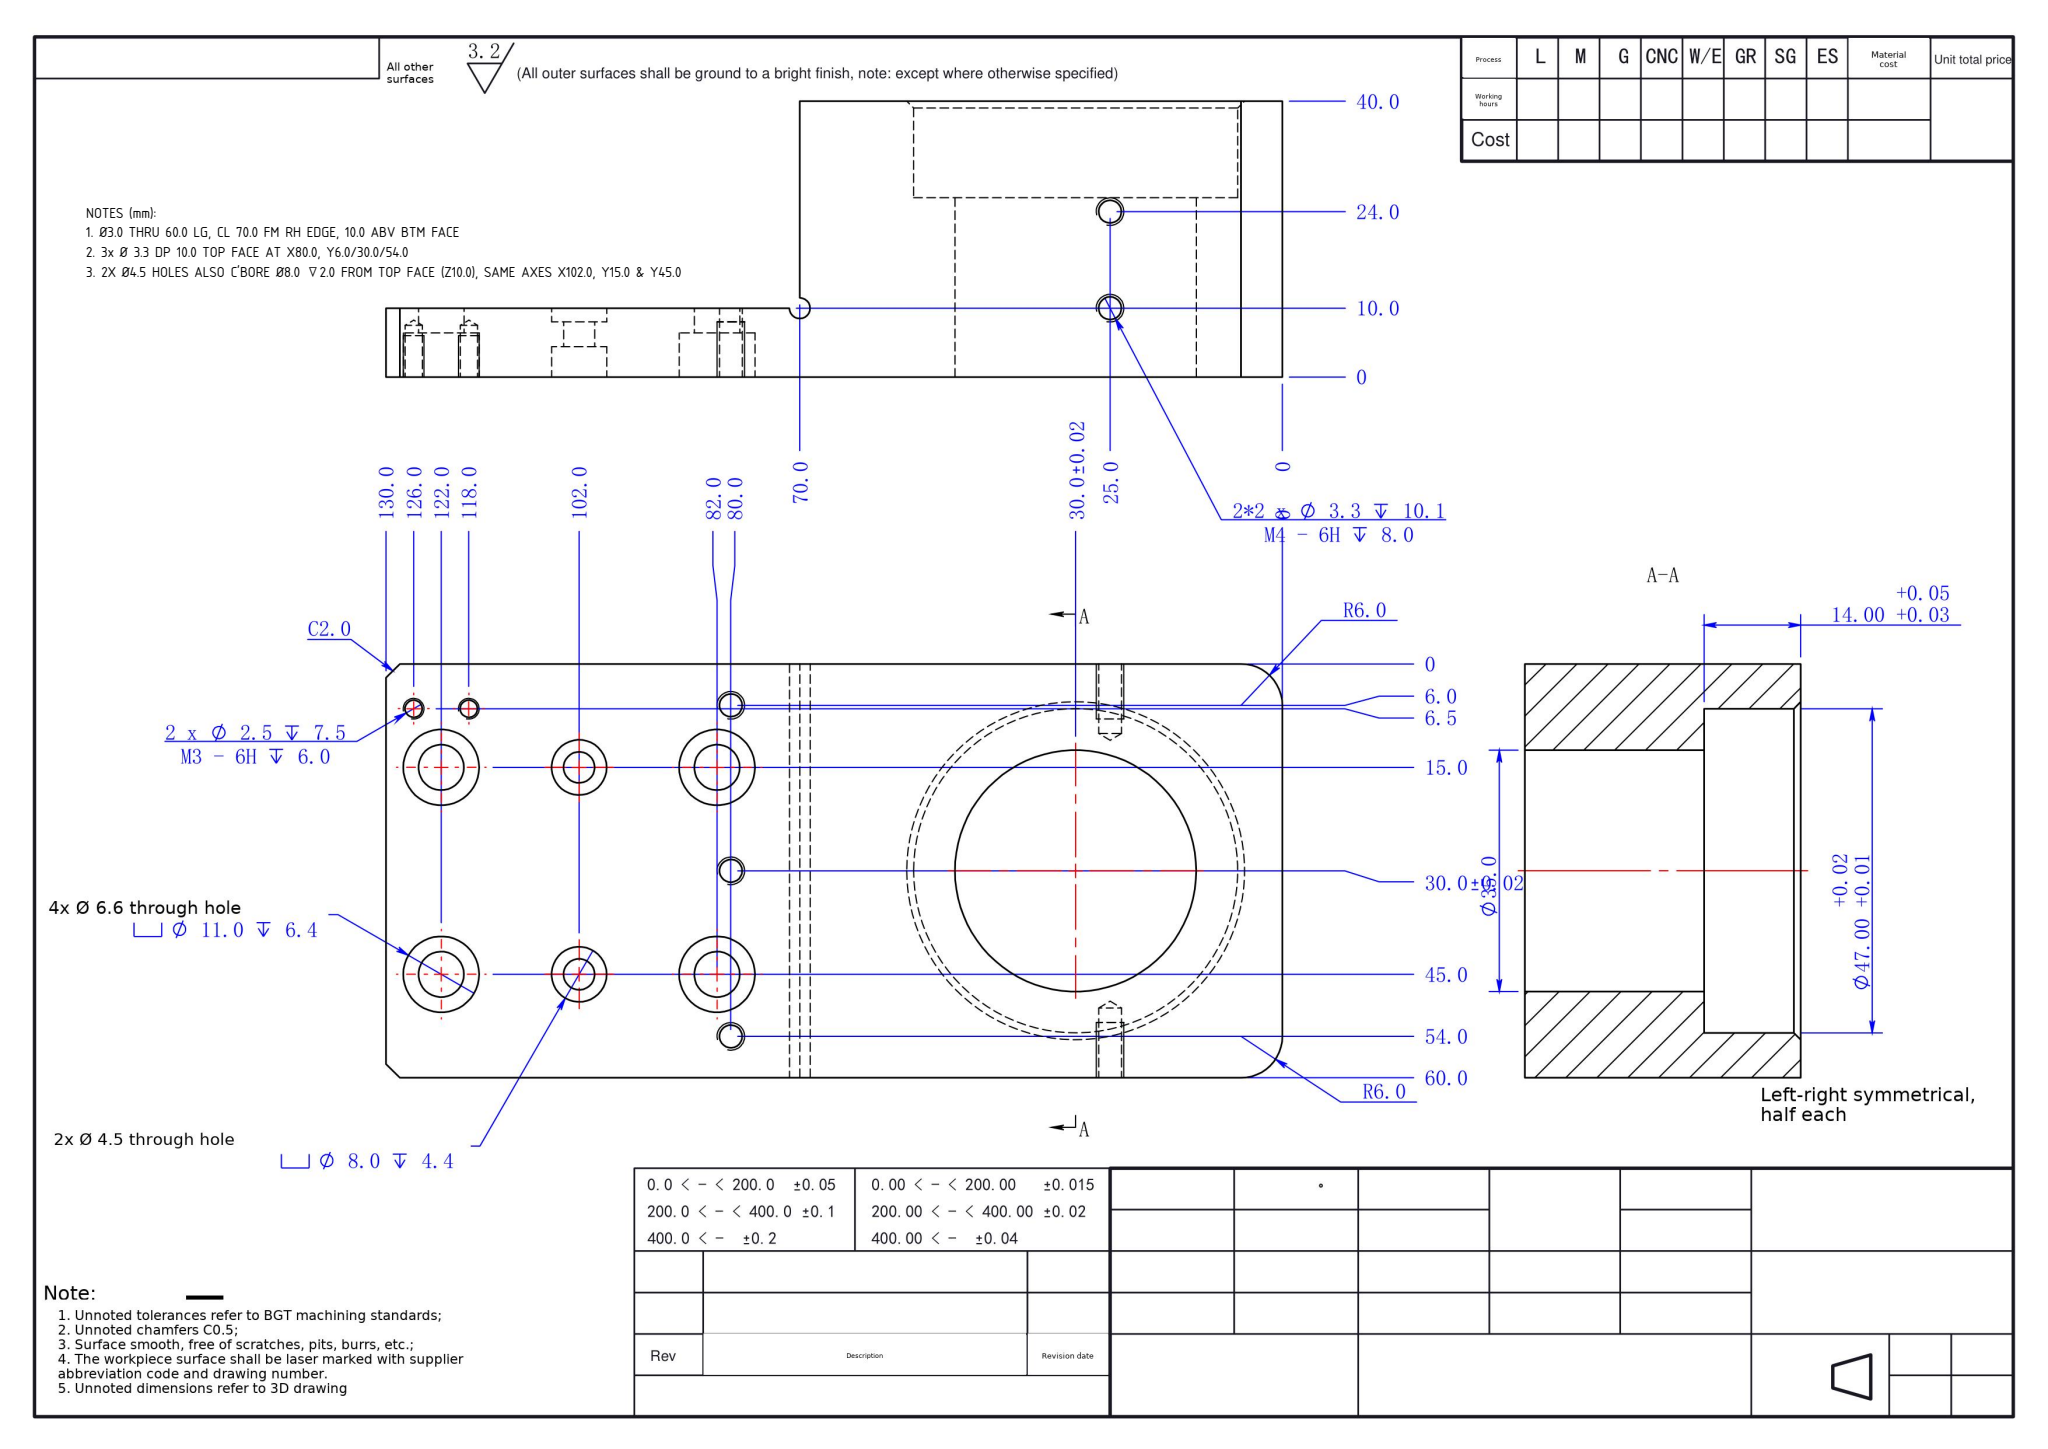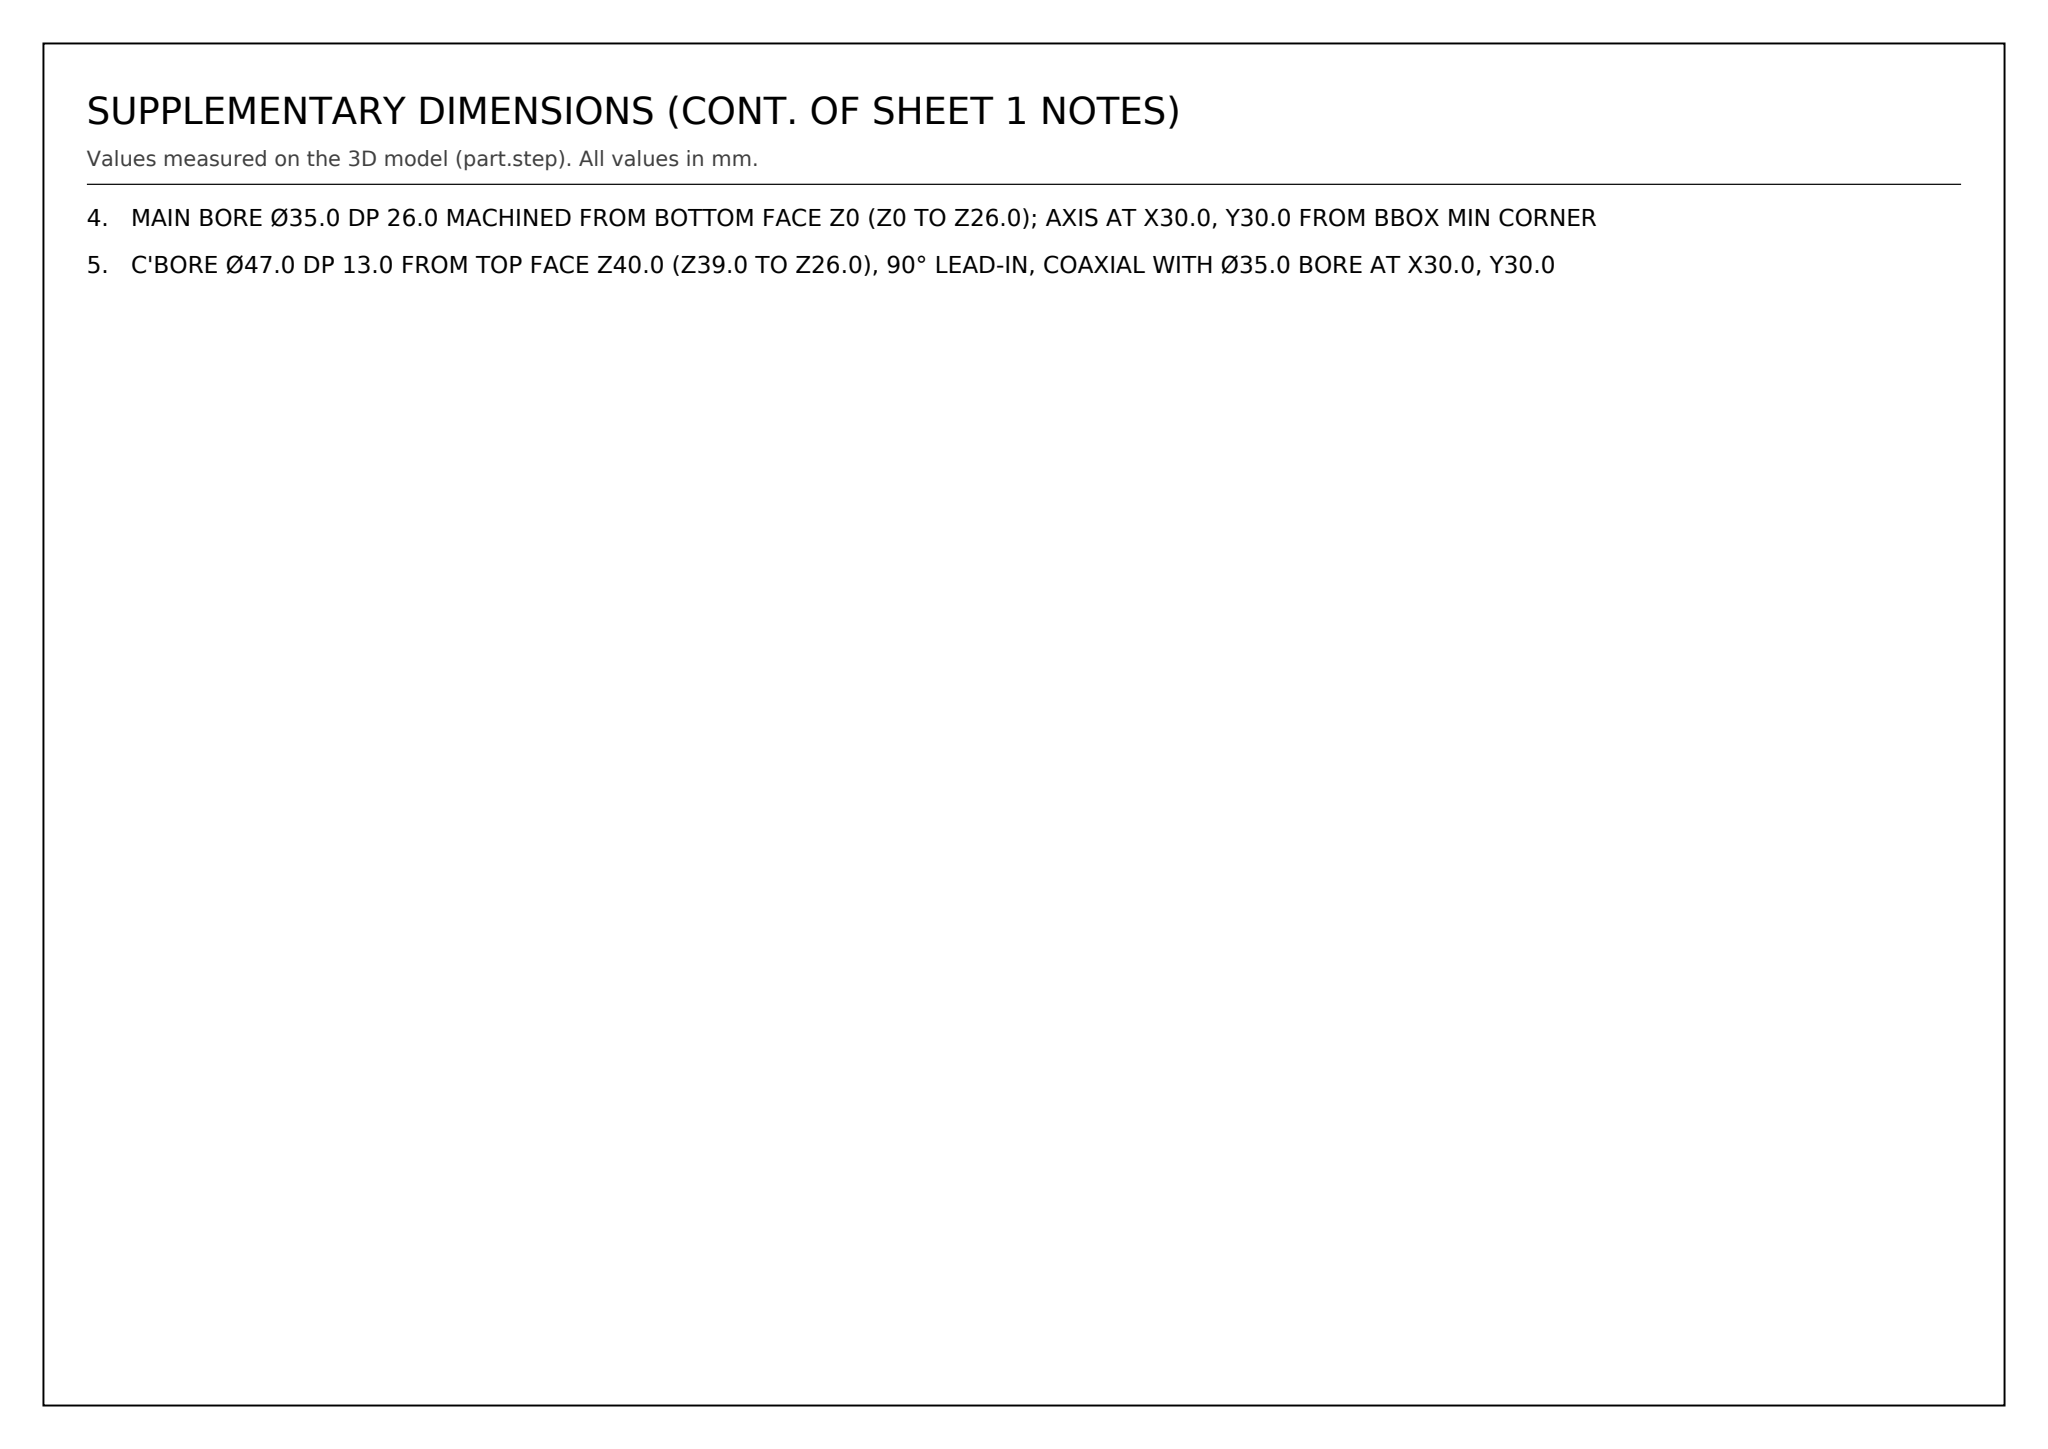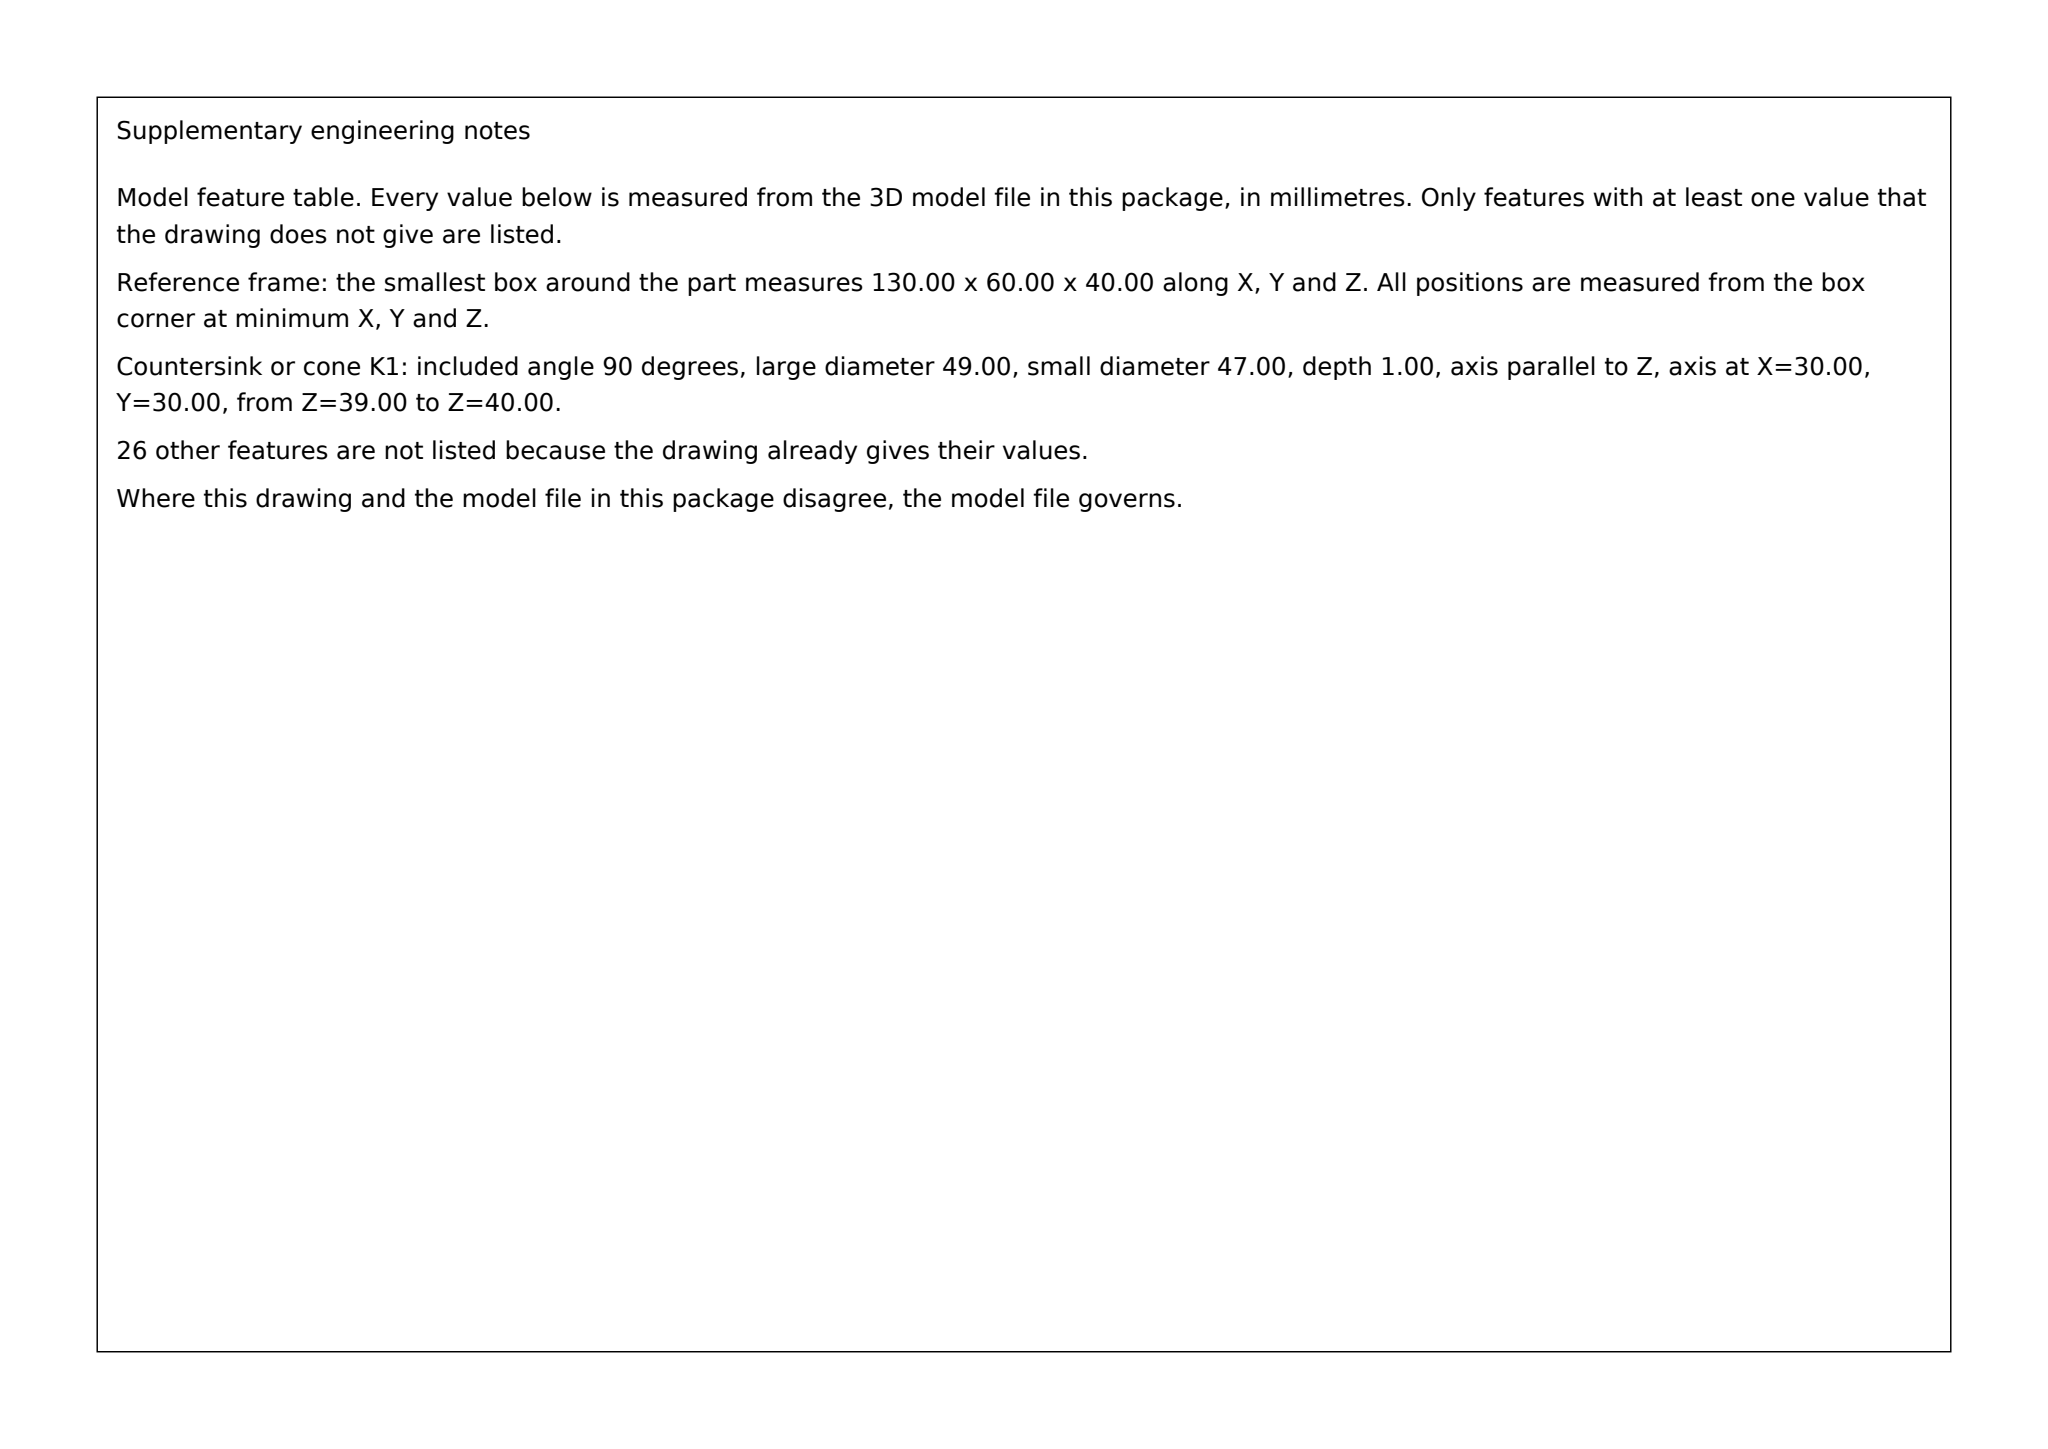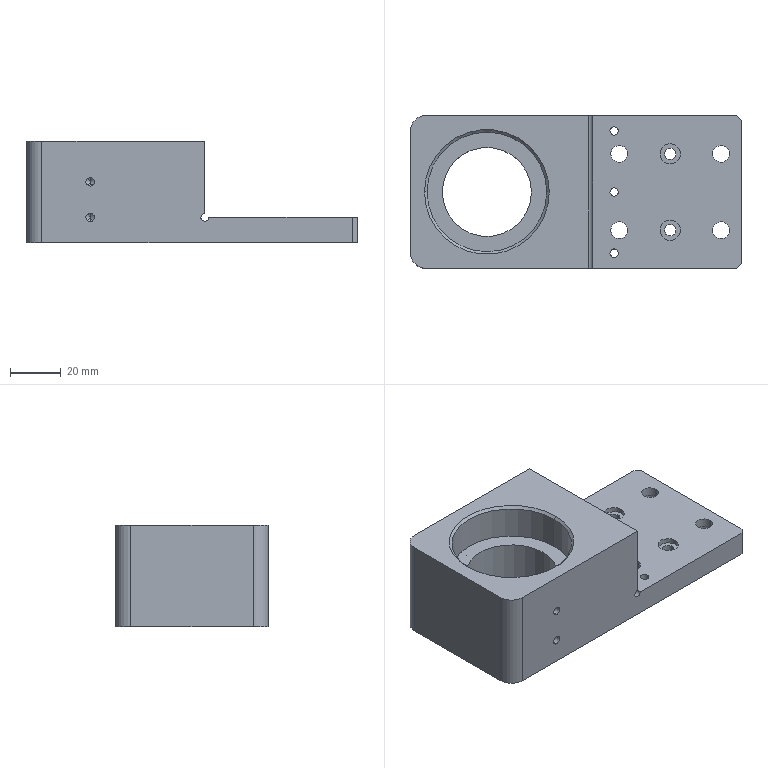Part | SolidWorks | mm | 1 solid | 86 faces | box 130 x 60 x 40 mm | volume 149272 mm3 | cylinder 53 | plane 19 | cone 14 | commonest cylinder face diameters 3.3 x14 8 x8 11 x8 6.6 x8 2.5 x4 4.5 x4 47 x2 35 x2
Drawing notes:
Ø3.0 THRU 60.0 LG, CL 70.0 FM RH EDGE, 10.0 ABV BTM FACE | from the solid: cylinder [3.0, axis y, pos x=70.0 z=10.0, length 60.0]
3x Ø 3.3 DP 10.0 TOP FACE AT X80.0, Y6.0/30.0/54.0 | from the solid: cylinders [3.3,"z",[80.0,6.0],10.0], [3.3,"z",[80.0,30.0],10.0], [3.3,"z",[80.0,54.0],10.0]; cone 118 deg ref dia 3.3 drill point
2X Ø4.5 HOLES ALSO C'BORE Ø8.0 ▽2.0 FROM TOP FACE (Z10.0), SAME AXES X102.0, Y15.0 & Y45.0 | from the solid: cylinders [8.0,z,(102,15),2.0] and [8.0,z,(102,45),2.0]; axis_plane z=8.0 count 2
MAIN BORE Ø35.0 DP 26.0 MACHINED FROM BOTTOM FACE Z0 (Z0 TO Z26.0); AXIS AT X30.0, Y30.0 FROM BBOX MIN CORNER | from the solid: cylinders: hole/bore dia 35.0, axis z at (30.0, 30.0), from 0.0 to 26.0
C'BORE Ø47.0 DP 13.0 FROM TOP FACE Z40.0 (Z39.0 TO Z26.0), 90° LEAD-IN, COAXIAL WITH Ø35.0 BORE AT X30.0, Y30.0 | from the solid: cylinders: hole/bore dia 47.0, axis z at (30.0, 30.0), from 26.0 to 39.0; cones: 90° included angle, ref dia 47.0
build123d program:
from build123d import *

# Parameters (mm, degrees)
SKETCH1_W                                       = 130
SKETCH1_H                                       = 60
BOSS_EXTRUDE1_DEPTH                             = 40
SKETCH2_W                                       = 60
SKETCH2_H                                       = 30
CUT_EXTRUDE1_DEPTH                              = 98.082
SKETCH3_R                                       = 17.5
CUT_EXTRUDE2_DEPTH                              = 83.006
FILLET1_R                                       = 6
SKETCH5_R                                       = 23.5
CUT_EXTRUDE3_DEPTH                              = 14
FILLET2_R                                       = 6
M6_HEX_SOCKET_HEAD_CAP_SCREW_CBORE1_D           = 6.6
M6_HEX_SOCKET_HEAD_CAP_SCREW_CBORE1_CBORE_D     = 11
M6_HEX_SOCKET_HEAD_CAP_SCREW_CBORE1_CBORE_DEPTH = 6.4
CHAMFER1_SIZE                                   = 2
M4_HEX_SOCKET_HEAD_CAP_SCREW_CBORE1_D           = 4.5
M4_HEX_SOCKET_HEAD_CAP_SCREW_CBORE1_CBORE_D     = 8
M4_HEX_SOCKET_HEAD_CAP_SCREW_CBORE1_CBORE_DEPTH = 4.4
CUT_EXTRUDE5_START                              = -2
SKETCH13_R                                      = 4
CUT_EXTRUDE5_DEPTH                              = 2
SKETCH14_R                                      = 1.5
CUT_EXTRUDE6_DEPTH                              = 98.082
CHAMFER2_SIZE                                   = 1
M3_TAPPED_HOLE1_D                               = 2.5
M3_TAPPED_HOLE1_DEPTH                           = 7.5
M3_TAPPED_HOLE1_TIP                             = 0.7511
M4_TAPPED_HOLE2_AT_2_COUNT                      = 2
M4_TAPPED_HOLE2_AT_2_PITCH                      = 14
M4_TAPPED_HOLE3_D                               = 3.3
M4_TAPPED_HOLE3_DEPTH                           = 10.1
M4_TAPPED_HOLE3_TIP                             = 0.9914


with BuildPart() as part:
    # Sketch1 → Boss-Extrude1 (new body)
    with BuildSketch(Plane.XY):
        Rectangle(SKETCH1_W, SKETCH1_H)
    extrude(amount=BOSS_EXTRUDE1_DEPTH)

    # Sketch2 → Cut-Extrude1 (cut, through all)
    with BuildSketch(Plane(origin=(0, 30, 0), x_dir=(1, 0, 0), z_dir=(0, 1, 0))):
        with Locations((35, -25)):
            Rectangle(SKETCH2_W, SKETCH2_H)
    extrude(amount=-CUT_EXTRUDE1_DEPTH, mode=Mode.SUBTRACT)

    # Sketch3 → Cut-Extrude2 (cut, through all)
    with BuildSketch(Plane.XY.offset(40)):
        with Locations((-35, 0)):
            Circle(SKETCH3_R)
    extrude(amount=-CUT_EXTRUDE2_DEPTH, mode=Mode.SUBTRACT)

    # Fillet1
    fillet1_edges = [part.edges().sort_by_distance(p)[0] for p in [
        (-65, -30, 20),
    ]]
    fillet(fillet1_edges, radius=FILLET1_R)

    # Sketch5 → Cut-Extrude3 (cut)
    with BuildSketch(Plane.XY.offset(40)):
        with Locations((-35, 0)):
            Circle(SKETCH5_R)
    extrude(amount=-CUT_EXTRUDE3_DEPTH, mode=Mode.SUBTRACT)

    # Fillet2
    fillet2_edges = [part.edges().sort_by_distance(p)[0] for p in [
        (-65, 30, 20),
    ]]
    fillet(fillet2_edges, radius=FILLET2_R)

    # M6 Hex Socket Head Cap Screw CBORE1 (through all)
    with Locations(Plane(origin=(0, 0, 0), x_dir=(-1, 0, 0), z_dir=(0, 0, -1))):
        with Locations((-57, 15), (-17, 15), (-17, -15), (-57, -15)):
            CounterBoreHole(M6_HEX_SOCKET_HEAD_CAP_SCREW_CBORE1_D / 2, M6_HEX_SOCKET_HEAD_CAP_SCREW_CBORE1_CBORE_D / 2, M6_HEX_SOCKET_HEAD_CAP_SCREW_CBORE1_CBORE_DEPTH)

    # Chamfer1
    chamfer1_edges = [part.edges().sort_by_distance(p)[0] for p in [
        (65, -30, 5),
        (65, 30, 5),
    ]]
    chamfer(chamfer1_edges, length=CHAMFER1_SIZE)

    # M4 Hex Socket Head Cap Screw CBORE1 (through all)
    with Locations(Plane(origin=(0, 0, 0), x_dir=(-1, 0, 0), z_dir=(0, 0, -1))):
        with Locations((-37, 15), (-37, -15)):
            CounterBoreHole(M4_HEX_SOCKET_HEAD_CAP_SCREW_CBORE1_D / 2, M4_HEX_SOCKET_HEAD_CAP_SCREW_CBORE1_CBORE_D / 2, M4_HEX_SOCKET_HEAD_CAP_SCREW_CBORE1_CBORE_DEPTH)

    # Sketch13 → Cut-Extrude5 (cut)
    with BuildSketch(Plane.XY.offset(10).offset(CUT_EXTRUDE5_START)):
        with Locations(Location((37, 15, 0), (0, 0, 180))):
            Circle(SKETCH13_R)
        with Locations(Location((37, -15, 0), (0, 0, 180))):
            Circle(SKETCH13_R)
    extrude(amount=CUT_EXTRUDE5_DEPTH, mode=Mode.SUBTRACT)

    # Sketch14 → Cut-Extrude6 (cut, through all)
    with BuildSketch(Plane(origin=(0, 30, 0), x_dir=(1, 0, 0), z_dir=(0, 1, 0))):
        with Locations((5, -10)):
            Circle(SKETCH14_R)
    extrude(amount=-CUT_EXTRUDE6_DEPTH, mode=Mode.SUBTRACT)

    # Chamfer2
    chamfer2_edges = [part.edges().sort_by_distance(p)[0] for p in [
        (-58.5, 0, 40),
    ]]
    chamfer(chamfer2_edges, length=CHAMFER2_SIZE)

    # M3 Tapped Hole1
    with Locations(Plane(origin=(0, 0, 0), x_dir=(-1, 0, 0), z_dir=(0, 0, -1))):
        with Locations((-53, 23.5), (-61, 23.5)):
            Hole(M3_TAPPED_HOLE1_D / 2, depth=M3_TAPPED_HOLE1_DEPTH)
            with Locations((0, 0, -(M3_TAPPED_HOLE1_DEPTH + M3_TAPPED_HOLE1_TIP / 2))):  # 118° drill point
                Cone(0, M3_TAPPED_HOLE1_D / 2, M3_TAPPED_HOLE1_TIP, mode=Mode.SUBTRACT)

    # Sketch18 → M4 Tapped Hole2 (revolve, cut)
    with BuildSketch(Plane(origin=(-40, 30, 10), x_dir=(0, 0, 1), z_dir=(1, 0, 0))):
        Polygon((0, 0), (0, 11.091), (1.65, 10.1), (1.65, 0), align=None)
    m4_tapped_hole2 = revolve(axis=Axis((-40, 36.35, 10), (0, -1, 0)), mode=Mode.SUBTRACT)

    # M4 Tapped Hole2 at 2: M4 Tapped Hole2 ×2
    with Locations(*[(0, 0, i * M4_TAPPED_HOLE2_AT_2_PITCH) for i in range(1, M4_TAPPED_HOLE2_AT_2_COUNT)]):
        add(m4_tapped_hole2, mode=Mode.SUBTRACT)

    # Mirror1: M4 Tapped Hole2 across plane
    add(m4_tapped_hole2.mirror(Plane.ZX), mode=Mode.SUBTRACT)

    # Mirror1 copy 1 sketch → Mirror1 copy 1 (revolve, cut)
    with BuildSketch(Plane(origin=(-40, -30, 24), x_dir=(0, 0, 1), z_dir=(1, 0, 0))):
        Polygon((0, 0), (0, -11.091), (1.65, -10.1), (1.65, 0), align=None)
    revolve(axis=Axis((-40, -36.35, 24), (0, -1, 0)), mode=Mode.SUBTRACT)

    # M4 Tapped Hole3
    with Locations(Plane(origin=(0, 0, 0), x_dir=(-1, 0, 0), z_dir=(0, 0, -1))):
        with Locations((-15, 24), (-15, 0), (-15, -24)):
            Hole(M4_TAPPED_HOLE3_D / 2, depth=M4_TAPPED_HOLE3_DEPTH)
            with Locations((0, 0, -(M4_TAPPED_HOLE3_DEPTH + M4_TAPPED_HOLE3_TIP / 2))):  # 118° drill point
                Cone(0, M4_TAPPED_HOLE3_D / 2, M4_TAPPED_HOLE3_TIP, mode=Mode.SUBTRACT)


solid = part.part